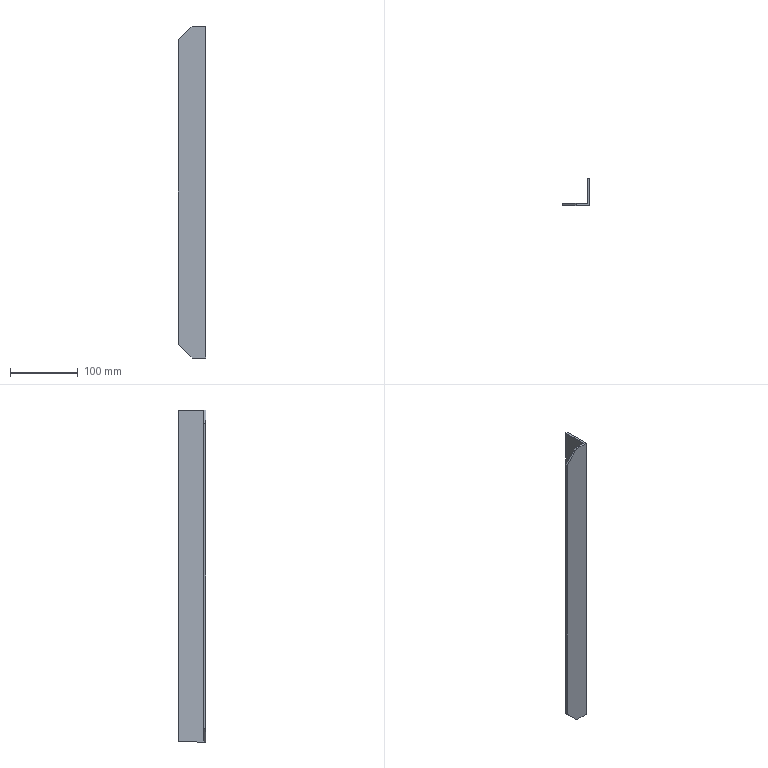Component | SolidWorks | LX-TSJ-15-2 | 1 solid | 10 faces | box 40 x 40 x 490 mm | volume 111990 mm3 | plane 10
STEP:
#1=CARTESIAN_POINT('',(-15.473,-25.051,-26.153));
#2=VERTEX_POINT('',#1);
#3=CARTESIAN_POINT('',(-15.473,-25.051,-6.862));
#4=VERTEX_POINT('',#3);
#5=CARTESIAN_POINT('',(-15.473,-25.051,-26.153));
#6=DIRECTION('',(0.,-0.,1.));
#7=VECTOR('',#6,39.37);
#8=LINE('',#5,#7);
#9=EDGE_CURVE('',#2,#4,#8,.T.);
#10=ORIENTED_EDGE('',*,*,#9,.F.);
#11=CARTESIAN_POINT('',(-15.473,-23.476,-26.153));
#12=VERTEX_POINT('',#11);
#13=CARTESIAN_POINT('',(-15.473,-25.051,-26.153));
#14=DIRECTION('',(-0.,-1.,-0.));
#15=VECTOR('',#14,39.37);
#16=LINE('',#13,#15);
#17=EDGE_CURVE('',#12,#2,#16,.T.);
#18=ORIENTED_EDGE('',*,*,#17,.F.);
#19=CARTESIAN_POINT('',(-15.473,-23.476,-6.862));
#20=VERTEX_POINT('',#19);
#21=CARTESIAN_POINT('',(-15.473,-23.476,-26.153));
#22=DIRECTION('',(0.,0.,-1.));
#23=VECTOR('',#22,39.37);
#24=LINE('',#21,#23);
#25=EDGE_CURVE('',#20,#12,#24,.T.);
#26=ORIENTED_EDGE('',*,*,#25,.F.);
#27=CARTESIAN_POINT('',(-15.473,-25.051,-6.862));
#28=DIRECTION('',(0.,1.,0.));
#29=VECTOR('',#28,39.37);
#30=LINE('',#27,#29);
#31=EDGE_CURVE('',#4,#20,#30,.T.);
#32=ORIENTED_EDGE('',*,*,#31,.F.);
#33=EDGE_LOOP('',(#10,#18,#26,#32));
#34=FACE_OUTER_BOUND('',#33,.T.);
#35=CARTESIAN_POINT('',(-15.473,-25.051,-26.153));
#36=DIRECTION('',(-1.,0.,0.));
#37=DIRECTION('',(0.,0.,-1.));
#38=AXIS2_PLACEMENT_3D('',#35,#36,#37);
#39=PLANE('',#38);
#40=ADVANCED_FACE('',(#34),#39,.F.);
#41=CARTESIAN_POINT('',(-15.591,-24.933,-6.862));
#42=VERTEX_POINT('',#41);
#43=CARTESIAN_POINT('',(-15.591,-23.476,-6.862));
#44=VERTEX_POINT('',#43);
#45=CARTESIAN_POINT('',(-15.591,-25.051,-6.862));
#46=DIRECTION('',(0.,1.,0.));
#47=VECTOR('',#46,39.37);
#48=LINE('',#45,#47);
#49=EDGE_CURVE('',#42,#44,#48,.T.);
#50=ORIENTED_EDGE('',*,*,#49,.F.);
#51=CARTESIAN_POINT('',(-16.261,-24.933,-6.862));
#52=VERTEX_POINT('',#51);
#53=CARTESIAN_POINT('',(-17.048,-24.933,-6.862));
#54=DIRECTION('',(1.,-0.,-0.));
#55=VECTOR('',#54,39.37);
#56=LINE('',#53,#55);
#57=EDGE_CURVE('',#52,#42,#56,.T.);
#58=ORIENTED_EDGE('',*,*,#57,.F.);
#59=CARTESIAN_POINT('',(-16.261,-25.051,-6.862));
#60=VERTEX_POINT('',#59);
#61=CARTESIAN_POINT('',(-16.261,-25.051,-6.862));
#62=DIRECTION('',(0.,1.,0.));
#63=VECTOR('',#62,39.37);
#64=LINE('',#61,#63);
#65=EDGE_CURVE('',#60,#52,#64,.T.);
#66=ORIENTED_EDGE('',*,*,#65,.F.);
#67=CARTESIAN_POINT('',(-17.048,-25.051,-6.862));
#68=DIRECTION('',(-1.,0.,0.));
#69=VECTOR('',#68,39.37);
#70=LINE('',#67,#69);
#71=EDGE_CURVE('',#4,#60,#70,.T.);
#72=ORIENTED_EDGE('',*,*,#71,.F.);
#73=ORIENTED_EDGE('',*,*,#31,.T.);
#74=CARTESIAN_POINT('',(-17.048,-23.476,-6.862));
#75=DIRECTION('',(1.,-0.,-0.));
#76=VECTOR('',#75,39.37);
#77=LINE('',#74,#76);
#78=EDGE_CURVE('',#44,#20,#77,.T.);
#79=ORIENTED_EDGE('',*,*,#78,.F.);
#80=EDGE_LOOP('',(#50,#58,#66,#72,#73,#79));
#81=FACE_OUTER_BOUND('',#80,.T.);
#82=CARTESIAN_POINT('',(-17.048,-25.051,-6.862));
#83=DIRECTION('',(0.,0.,-1.));
#84=DIRECTION('',(1.,-0.,-0.));
#85=AXIS2_PLACEMENT_3D('',#82,#83,#84);
#86=PLANE('',#85);
#87=ADVANCED_FACE('',(#81),#86,.F.);
#88=ORIENTED_EDGE('',*,*,#71,.T.);
#89=CARTESIAN_POINT('',(-17.048,-25.051,-7.65));
#90=VERTEX_POINT('',#89);
#91=CARTESIAN_POINT('',(-17.048,-25.051,-7.65));
#92=DIRECTION('',(0.7071,-0.,0.7071));
#93=VECTOR('',#92,39.37);
#94=LINE('',#91,#93);
#95=EDGE_CURVE('',#90,#60,#94,.T.);
#96=ORIENTED_EDGE('',*,*,#95,.F.);
#97=CARTESIAN_POINT('',(-17.048,-25.051,-25.366));
#98=VERTEX_POINT('',#97);
#99=CARTESIAN_POINT('',(-17.048,-25.051,-26.153));
#100=DIRECTION('',(0.,-0.,1.));
#101=VECTOR('',#100,39.37);
#102=LINE('',#99,#101);
#103=EDGE_CURVE('',#98,#90,#102,.T.);
#104=ORIENTED_EDGE('',*,*,#103,.F.);
#105=CARTESIAN_POINT('',(-16.261,-25.051,-26.153));
#106=VERTEX_POINT('',#105);
#107=CARTESIAN_POINT('',(-16.261,-25.051,-26.153));
#108=DIRECTION('',(-0.7071,-0.,0.7071));
#109=VECTOR('',#108,39.37);
#110=LINE('',#107,#109);
#111=EDGE_CURVE('',#106,#98,#110,.T.);
#112=ORIENTED_EDGE('',*,*,#111,.F.);
#113=CARTESIAN_POINT('',(-17.048,-25.051,-26.153));
#114=DIRECTION('',(-1.,0.,0.));
#115=VECTOR('',#114,39.37);
#116=LINE('',#113,#115);
#117=EDGE_CURVE('',#2,#106,#116,.T.);
#118=ORIENTED_EDGE('',*,*,#117,.F.);
#119=ORIENTED_EDGE('',*,*,#9,.T.);
#120=EDGE_LOOP('',(#88,#96,#104,#112,#118,#119));
#121=FACE_OUTER_BOUND('',#120,.T.);
#122=CARTESIAN_POINT('',(-17.048,-25.051,-26.153));
#123=DIRECTION('',(0.,1.,0.));
#124=DIRECTION('',(0.,-0.,1.));
#125=AXIS2_PLACEMENT_3D('',#122,#123,#124);
#126=PLANE('',#125);
#127=ADVANCED_FACE('',(#121),#126,.F.);
#128=ORIENTED_EDGE('',*,*,#117,.T.);
#129=CARTESIAN_POINT('',(-16.261,-24.933,-26.153));
#130=VERTEX_POINT('',#129);
#131=CARTESIAN_POINT('',(-16.261,-25.051,-26.153));
#132=DIRECTION('',(0.,1.,0.));
#133=VECTOR('',#132,39.37);
#134=LINE('',#131,#133);
#135=EDGE_CURVE('',#106,#130,#134,.T.);
#136=ORIENTED_EDGE('',*,*,#135,.T.);
#137=CARTESIAN_POINT('',(-15.591,-24.933,-26.153));
#138=VERTEX_POINT('',#137);
#139=CARTESIAN_POINT('',(-17.048,-24.933,-26.153));
#140=DIRECTION('',(1.,-0.,-0.));
#141=VECTOR('',#140,39.37);
#142=LINE('',#139,#141);
#143=EDGE_CURVE('',#130,#138,#142,.T.);
#144=ORIENTED_EDGE('',*,*,#143,.T.);
#145=CARTESIAN_POINT('',(-15.591,-23.476,-26.153));
#146=VERTEX_POINT('',#145);
#147=CARTESIAN_POINT('',(-15.591,-25.051,-26.153));
#148=DIRECTION('',(0.,1.,0.));
#149=VECTOR('',#148,39.37);
#150=LINE('',#147,#149);
#151=EDGE_CURVE('',#138,#146,#150,.T.);
#152=ORIENTED_EDGE('',*,*,#151,.T.);
#153=CARTESIAN_POINT('',(-17.048,-23.476,-26.153));
#154=DIRECTION('',(1.,-0.,-0.));
#155=VECTOR('',#154,39.37);
#156=LINE('',#153,#155);
#157=EDGE_CURVE('',#146,#12,#156,.T.);
#158=ORIENTED_EDGE('',*,*,#157,.T.);
#159=ORIENTED_EDGE('',*,*,#17,.T.);
#160=EDGE_LOOP('',(#128,#136,#144,#152,#158,#159));
#161=FACE_OUTER_BOUND('',#160,.T.);
#162=CARTESIAN_POINT('',(-17.048,-25.051,-26.153));
#163=DIRECTION('',(0.,0.,-1.));
#164=DIRECTION('',(1.,-0.,-0.));
#165=AXIS2_PLACEMENT_3D('',#162,#163,#164);
#166=PLANE('',#165);
#167=ADVANCED_FACE('',(#161),#166,.T.);
#168=ORIENTED_EDGE('',*,*,#25,.T.);
#169=ORIENTED_EDGE('',*,*,#157,.F.);
#170=CARTESIAN_POINT('',(-15.591,-23.476,-26.153));
#171=DIRECTION('',(0.,0.,-1.));
#172=VECTOR('',#171,39.37);
#173=LINE('',#170,#172);
#174=EDGE_CURVE('',#44,#146,#173,.T.);
#175=ORIENTED_EDGE('',*,*,#174,.F.);
#176=ORIENTED_EDGE('',*,*,#78,.T.);
#177=EDGE_LOOP('',(#168,#169,#175,#176));
#178=FACE_OUTER_BOUND('',#177,.T.);
#179=CARTESIAN_POINT('',(-15.591,-23.476,-26.153));
#180=DIRECTION('',(-0.,-1.,-0.));
#181=DIRECTION('',(0.,0.,-1.));
#182=AXIS2_PLACEMENT_3D('',#179,#180,#181);
#183=PLANE('',#182);
#184=ADVANCED_FACE('',(#178),#183,.F.);
#185=CARTESIAN_POINT('',(-17.048,-24.933,-25.366));
#186=VERTEX_POINT('',#185);
#187=CARTESIAN_POINT('',(-17.048,-24.933,-25.366));
#188=DIRECTION('',(0.7071,0.,-0.7071));
#189=VECTOR('',#188,39.37);
#190=LINE('',#187,#189);
#191=EDGE_CURVE('',#186,#130,#190,.T.);
#192=ORIENTED_EDGE('',*,*,#191,.F.);
#193=CARTESIAN_POINT('',(-17.048,-24.933,-7.65));
#194=VERTEX_POINT('',#193);
#195=CARTESIAN_POINT('',(-17.048,-24.933,-26.153));
#196=DIRECTION('',(0.,0.,-1.));
#197=VECTOR('',#196,39.37);
#198=LINE('',#195,#197);
#199=EDGE_CURVE('',#194,#186,#198,.T.);
#200=ORIENTED_EDGE('',*,*,#199,.F.);
#201=CARTESIAN_POINT('',(-16.261,-24.933,-6.862));
#202=DIRECTION('',(-0.7071,0.,-0.7071));
#203=VECTOR('',#202,39.37);
#204=LINE('',#201,#203);
#205=EDGE_CURVE('',#52,#194,#204,.T.);
#206=ORIENTED_EDGE('',*,*,#205,.F.);
#207=ORIENTED_EDGE('',*,*,#57,.T.);
#208=CARTESIAN_POINT('',(-15.591,-24.933,-26.153));
#209=DIRECTION('',(0.,-0.,1.));
#210=VECTOR('',#209,39.37);
#211=LINE('',#208,#210);
#212=EDGE_CURVE('',#138,#42,#211,.T.);
#213=ORIENTED_EDGE('',*,*,#212,.F.);
#214=ORIENTED_EDGE('',*,*,#143,.F.);
#215=EDGE_LOOP('',(#192,#200,#206,#207,#213,#214));
#216=FACE_OUTER_BOUND('',#215,.T.);
#217=CARTESIAN_POINT('',(-17.048,-24.933,-26.153));
#218=DIRECTION('',(-0.,-1.,-0.));
#219=DIRECTION('',(0.,0.,-1.));
#220=AXIS2_PLACEMENT_3D('',#217,#218,#219);
#221=PLANE('',#220);
#222=ADVANCED_FACE('',(#216),#221,.F.);
#223=ORIENTED_EDGE('',*,*,#65,.T.);
#224=ORIENTED_EDGE('',*,*,#205,.T.);
#225=CARTESIAN_POINT('',(-17.048,-25.051,-7.65));
#226=DIRECTION('',(0.,1.,0.));
#227=VECTOR('',#226,39.37);
#228=LINE('',#225,#227);
#229=EDGE_CURVE('',#90,#194,#228,.T.);
#230=ORIENTED_EDGE('',*,*,#229,.F.);
#231=ORIENTED_EDGE('',*,*,#95,.T.);
#232=EDGE_LOOP('',(#223,#224,#230,#231));
#233=FACE_OUTER_BOUND('',#232,.T.);
#234=CARTESIAN_POINT('',(-17.048,-25.051,-7.65));
#235=DIRECTION('',(0.7071,0.,-0.7071));
#236=DIRECTION('',(0.7071,-0.,0.7071));
#237=AXIS2_PLACEMENT_3D('',#234,#235,#236);
#238=PLANE('',#237);
#239=ADVANCED_FACE('',(#233),#238,.F.);
#240=ORIENTED_EDGE('',*,*,#174,.T.);
#241=ORIENTED_EDGE('',*,*,#151,.F.);
#242=ORIENTED_EDGE('',*,*,#212,.T.);
#243=ORIENTED_EDGE('',*,*,#49,.T.);
#244=EDGE_LOOP('',(#240,#241,#242,#243));
#245=FACE_OUTER_BOUND('',#244,.T.);
#246=CARTESIAN_POINT('',(-15.591,-24.933,-26.153));
#247=DIRECTION('',(1.,-0.,-0.));
#248=DIRECTION('',(0.,-0.,1.));
#249=AXIS2_PLACEMENT_3D('',#246,#247,#248);
#250=PLANE('',#249);
#251=ADVANCED_FACE('',(#245),#250,.F.);
#252=CARTESIAN_POINT('',(-17.048,-25.051,-25.366));
#253=DIRECTION('',(0.,1.,0.));
#254=VECTOR('',#253,39.37);
#255=LINE('',#252,#254);
#256=EDGE_CURVE('',#98,#186,#255,.T.);
#257=ORIENTED_EDGE('',*,*,#256,.F.);
#258=ORIENTED_EDGE('',*,*,#103,.T.);
#259=ORIENTED_EDGE('',*,*,#229,.T.);
#260=ORIENTED_EDGE('',*,*,#199,.T.);
#261=EDGE_LOOP('',(#257,#258,#259,#260));
#262=FACE_OUTER_BOUND('',#261,.T.);
#263=CARTESIAN_POINT('',(-17.048,-25.051,-26.153));
#264=DIRECTION('',(1.,-0.,-0.));
#265=DIRECTION('',(0.,-0.,1.));
#266=AXIS2_PLACEMENT_3D('',#263,#264,#265);
#267=PLANE('',#266);
#268=ADVANCED_FACE('',(#262),#267,.F.);
#269=ORIENTED_EDGE('',*,*,#191,.T.);
#270=ORIENTED_EDGE('',*,*,#135,.F.);
#271=ORIENTED_EDGE('',*,*,#111,.T.);
#272=ORIENTED_EDGE('',*,*,#256,.T.);
#273=EDGE_LOOP('',(#269,#270,#271,#272));
#274=FACE_OUTER_BOUND('',#273,.T.);
#275=CARTESIAN_POINT('',(-16.261,-25.051,-26.153));
#276=DIRECTION('',(-0.7071,0.,-0.7071));
#277=DIRECTION('',(0.7071,0.,-0.7071));
#278=AXIS2_PLACEMENT_3D('',#275,#276,#277);
#279=PLANE('',#278);
#280=ADVANCED_FACE('',(#274),#279,.T.);
#281=CLOSED_SHELL('',(#40,#87,#127,#167,#184,#222,#239,#251,#268,#280));
#282=MANIFOLD_SOLID_BREP('',#281);
#283=CARTESIAN_POINT('',(0.,0.,0.));
#284=DIRECTION('',(0.,0.,1.));
#285=DIRECTION('',(1.,0.,0.));
#286=AXIS2_PLACEMENT_3D('',#283,#284,#285);
#287=(LENGTH_UNIT()NAMED_UNIT(*)SI_UNIT($,.METRE.));
#288=LENGTH_MEASURE_WITH_UNIT(LENGTH_MEASURE(0.0254),#287);
#289=DIMENSIONAL_EXPONENTS(1.,0.,0.,0.,0.,0.,0.);
#290=(CONVERSION_BASED_UNIT('',#288)LENGTH_UNIT()NAMED_UNIT(#289));
#291=UNCERTAINTY_MEASURE_WITH_UNIT(LENGTH_MEASURE(0.00001),#290,'','');
#292=(NAMED_UNIT(*)PLANE_ANGLE_UNIT()SI_UNIT($,.RADIAN.));
#293=(NAMED_UNIT(*)SI_UNIT($,.STERADIAN.)SOLID_ANGLE_UNIT());
#294=(GEOMETRIC_REPRESENTATION_CONTEXT(3)GLOBAL_UNCERTAINTY_ASSIGNED_CONTEXT((#291))GLOBAL_UNIT_ASSIGNED_CONTEXT((#290,#292,#293))REPRESENTATION_CONTEXT('',''));
#295=ADVANCED_BREP_SHAPE_REPRESENTATION('',(#282,#286),#294);
#296=COLOUR_RGB('',0.7922,0.8196,0.9333);
#297=FILL_AREA_STYLE_COLOUR('',#296);
#298=FILL_AREA_STYLE('',(#297));
#299=SURFACE_STYLE_FILL_AREA(#298);
#300=SURFACE_SIDE_STYLE('',(#299));
#301=SURFACE_STYLE_USAGE(.BOTH.,#300);
#302=PRESENTATION_STYLE_ASSIGNMENT((#301));
#303=STYLED_ITEM('',(#302),#282);
#304=(LENGTH_UNIT()NAMED_UNIT(*)SI_UNIT($,.METRE.));
#305=LENGTH_MEASURE_WITH_UNIT(LENGTH_MEASURE(0.0254),#304);
#306=DIMENSIONAL_EXPONENTS(1.,0.,0.,0.,0.,0.,0.);
#307=(CONVERSION_BASED_UNIT('',#305)LENGTH_UNIT()NAMED_UNIT(#306));
#308=UNCERTAINTY_MEASURE_WITH_UNIT(LENGTH_MEASURE(0.00001),#307,'','');
#309=(NAMED_UNIT(*)PLANE_ANGLE_UNIT()SI_UNIT($,.RADIAN.));
#310=(NAMED_UNIT(*)SI_UNIT($,.STERADIAN.)SOLID_ANGLE_UNIT());
#311=(GEOMETRIC_REPRESENTATION_CONTEXT(3)GLOBAL_UNCERTAINTY_ASSIGNED_CONTEXT((#308))GLOBAL_UNIT_ASSIGNED_CONTEXT((#307,#309,#310))REPRESENTATION_CONTEXT('',''));
#312=MECHANICAL_DESIGN_GEOMETRIC_PRESENTATION_REPRESENTATION('',(#303),#311);
#313=PRESENTATION_LAYER_ASSIGNMENT('','',(#303));